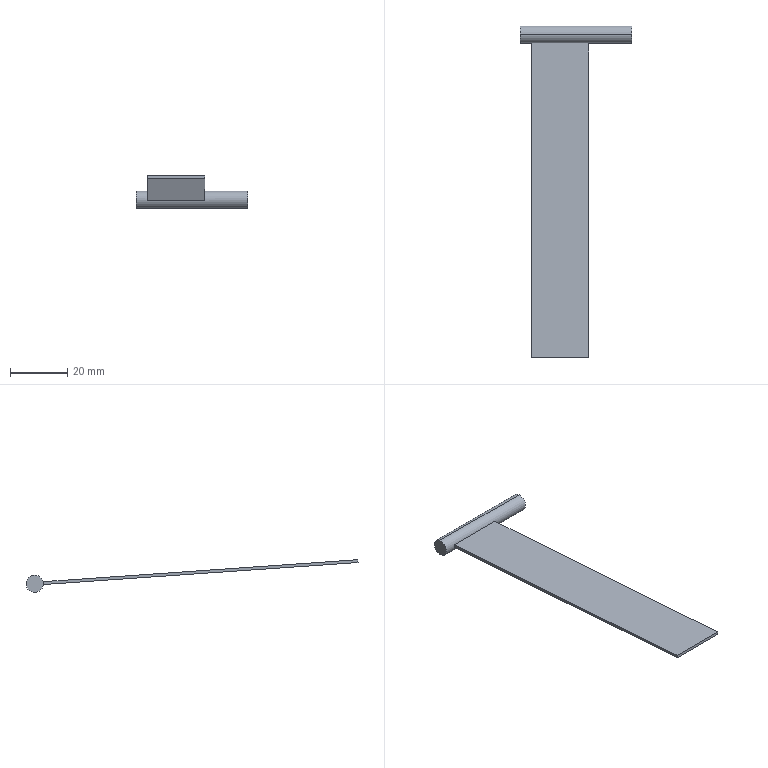Component | SolidWorks | OuterBagExpansionSheetMetalSidePlate-1 | 1 solid | 9 faces | box 39 x 115.72 x 11.36 mm | volume 3302 mm3 | plane 7 | cylinder 2 | commonest cylinder face diameters 6 x2
build123d program:
from build123d import *

# Parameters (mm, degrees)
SKETCH2_W                = 110
SKETCH2_H                = 20
BOSS_EXTRUDE1_DEPTH      = 1
BOSS_EXTRUDE2_DEPTH      = 4
BOSS_EXTRUDE2_DEPTH_BACK = 35
SKETCH3_R                = 3


with BuildPart() as part:
    # Sketch2 → Boss-Extrude1 (new body)
    with BuildSketch(Plane.XY):
        with Locations((-72.403, -7.81)):
            Rectangle(SKETCH2_W, SKETCH2_H)
    extrude(amount=BOSS_EXTRUDE1_DEPTH)

    # Sketch3 → Boss-Extrude2 (add, two sides: drawn at the far end of the back side and taken through both)
    with BuildSketch(Plane.XZ.offset(17.81).offset(-BOSS_EXTRUDE2_DEPTH_BACK)):
        with Locations(Location((-14.445, 0.5, 0), (0, 0, 270))):
            Circle(SKETCH3_R)
    extrude(amount=BOSS_EXTRUDE2_DEPTH + BOSS_EXTRUDE2_DEPTH_BACK)


solid = part.part

# Placed as in the assembly
solid = solid.moved(Location((-530.636, 26.871, 401.647), (176.009, 0, -90)))
STEP:
#1=COLOUR_RGB('',0.7922,0.8196,0.9333);
#2=FILL_AREA_STYLE_COLOUR('',#1);
#3=FILL_AREA_STYLE('',(#2));
#4=SURFACE_STYLE_FILL_AREA(#3);
#5=SURFACE_SIDE_STYLE('',(#4));
#6=SURFACE_STYLE_USAGE(.BOTH.,#5);
#7=PRESENTATION_STYLE_ASSIGNMENT((#6));
#8=CARTESIAN_POINT('',(-21.75,0.4975,15.951));
#9=VERTEX_POINT('',#8);
#10=CARTESIAN_POINT('',(-21.75,0.481,15.715));
#11=VERTEX_POINT('',#10);
#12=CARTESIAN_POINT('',(-21.75,0.4892,15.833));
#13=DIRECTION('',(-1.,0.,0.));
#14=DIRECTION('',(0.,0.0696,0.9976));
#15=AXIS2_PLACEMENT_3D('',#12,#13,#14);
#16=CIRCLE('',#15,0.1181);
#17=EDGE_CURVE('',#9,#11,#16,.T.);
#18=ORIENTED_EDGE('',*,*,#17,.F.);
#19=CARTESIAN_POINT('',(-20.214,0.4975,15.951));
#20=VERTEX_POINT('',#19);
#21=CARTESIAN_POINT('',(-21.75,0.4975,15.951));
#22=DIRECTION('',(1.,-0.,-0.));
#23=VECTOR('',#22,39.37);
#24=LINE('',#21,#23);
#25=EDGE_CURVE('',#9,#20,#24,.T.);
#26=ORIENTED_EDGE('',*,*,#25,.T.);
#27=CARTESIAN_POINT('',(-20.214,0.481,15.715));
#28=VERTEX_POINT('',#27);
#29=CARTESIAN_POINT('',(-20.214,0.4892,15.833));
#30=DIRECTION('',(-1.,0.,0.));
#31=DIRECTION('',(0.,0.0696,0.9976));
#32=AXIS2_PLACEMENT_3D('',#29,#30,#31);
#33=CIRCLE('',#32,0.1181);
#34=EDGE_CURVE('',#20,#28,#33,.T.);
#35=ORIENTED_EDGE('',*,*,#34,.T.);
#36=CARTESIAN_POINT('',(-21.75,0.481,15.715));
#37=DIRECTION('',(1.,-0.,-0.));
#38=VECTOR('',#37,39.37);
#39=LINE('',#36,#38);
#40=EDGE_CURVE('',#11,#28,#39,.T.);
#41=ORIENTED_EDGE('',*,*,#40,.F.);
#42=EDGE_LOOP('',(#18,#26,#35,#41));
#43=FACE_OUTER_BOUND('',#42,.T.);
#44=CARTESIAN_POINT('',(-21.75,0.4892,15.833));
#45=DIRECTION('',(1.,-0.,-0.));
#46=DIRECTION('',(0.,-0.0696,-0.9976));
#47=AXIS2_PLACEMENT_3D('',#44,#45,#46);
#48=CYLINDRICAL_SURFACE('',#47,0.1181);
#49=ADVANCED_FACE('',(#43),#48,.T.);
#50=CARTESIAN_POINT('',(-20.805,-3.946,16.162));
#51=VERTEX_POINT('',#50);
#52=CARTESIAN_POINT('',(-21.592,-3.946,16.162));
#53=VERTEX_POINT('',#52);
#54=CARTESIAN_POINT('',(-20.805,-3.946,16.162));
#55=DIRECTION('',(-1.,0.,0.));
#56=VECTOR('',#55,39.37);
#57=LINE('',#54,#56);
#58=EDGE_CURVE('',#51,#53,#57,.T.);
#59=ORIENTED_EDGE('',*,*,#58,.T.);
#60=CARTESIAN_POINT('',(-21.592,-3.949,16.123));
#61=VERTEX_POINT('',#60);
#62=CARTESIAN_POINT('',(-21.592,-3.949,16.123));
#63=DIRECTION('',(0.,0.0696,0.9976));
#64=VECTOR('',#63,39.37);
#65=LINE('',#62,#64);
#66=EDGE_CURVE('',#61,#53,#65,.T.);
#67=ORIENTED_EDGE('',*,*,#66,.F.);
#68=CARTESIAN_POINT('',(-20.805,-3.949,16.123));
#69=VERTEX_POINT('',#68);
#70=CARTESIAN_POINT('',(-20.805,-3.949,16.123));
#71=DIRECTION('',(-1.,0.,0.));
#72=VECTOR('',#71,39.37);
#73=LINE('',#70,#72);
#74=EDGE_CURVE('',#69,#61,#73,.T.);
#75=ORIENTED_EDGE('',*,*,#74,.F.);
#76=CARTESIAN_POINT('',(-20.805,-3.949,16.123));
#77=DIRECTION('',(0.,0.0696,0.9976));
#78=VECTOR('',#77,39.37);
#79=LINE('',#76,#78);
#80=EDGE_CURVE('',#69,#51,#79,.T.);
#81=ORIENTED_EDGE('',*,*,#80,.T.);
#82=EDGE_LOOP('',(#59,#67,#75,#81));
#83=FACE_OUTER_BOUND('',#82,.T.);
#84=CARTESIAN_POINT('',(-20.805,-3.949,16.123));
#85=DIRECTION('',(-0.,0.9976,-0.0696));
#86=DIRECTION('',(0.,0.0696,0.9976));
#87=AXIS2_PLACEMENT_3D('',#84,#85,#86);
#88=PLANE('',#87);
#89=ADVANCED_FACE('',(#83),#88,.F.);
#90=CARTESIAN_POINT('',(-21.592,0.3717,15.821));
#91=VERTEX_POINT('',#90);
#92=CARTESIAN_POINT('',(-21.592,0.3744,15.861));
#93=VERTEX_POINT('',#92);
#94=CARTESIAN_POINT('',(-21.592,0.4892,15.833));
#95=DIRECTION('',(-1.,0.,0.));
#96=DIRECTION('',(0.,-0.0696,-0.9976));
#97=AXIS2_PLACEMENT_3D('',#94,#95,#96);
#98=CIRCLE('',#97,0.1181);
#99=EDGE_CURVE('',#91,#93,#98,.T.);
#100=ORIENTED_EDGE('',*,*,#99,.F.);
#101=CARTESIAN_POINT('',(-21.592,-3.949,16.123));
#102=DIRECTION('',(-0.,0.9976,-0.0696));
#103=VECTOR('',#102,39.37);
#104=LINE('',#101,#103);
#105=EDGE_CURVE('',#61,#91,#104,.T.);
#106=ORIENTED_EDGE('',*,*,#105,.F.);
#107=ORIENTED_EDGE('',*,*,#66,.T.);
#108=CARTESIAN_POINT('',(-21.592,-3.946,16.162));
#109=DIRECTION('',(-0.,0.9976,-0.0696));
#110=VECTOR('',#109,39.37);
#111=LINE('',#108,#110);
#112=EDGE_CURVE('',#53,#93,#111,.T.);
#113=ORIENTED_EDGE('',*,*,#112,.T.);
#114=EDGE_LOOP('',(#100,#106,#107,#113));
#115=FACE_OUTER_BOUND('',#114,.T.);
#116=CARTESIAN_POINT('',(-21.592,-3.949,16.123));
#117=DIRECTION('',(1.,-0.,-0.));
#118=DIRECTION('',(-0.,-0.0696,-0.9976));
#119=AXIS2_PLACEMENT_3D('',#116,#117,#118);
#120=PLANE('',#119);
#121=ADVANCED_FACE('',(#115),#120,.F.);
#122=CARTESIAN_POINT('',(-20.805,0.3744,15.861));
#123=VERTEX_POINT('',#122);
#124=CARTESIAN_POINT('',(-20.805,0.3717,15.821));
#125=VERTEX_POINT('',#124);
#126=CARTESIAN_POINT('',(-20.805,0.4892,15.833));
#127=DIRECTION('',(1.,-0.,-0.));
#128=DIRECTION('',(0.,0.0696,0.9976));
#129=AXIS2_PLACEMENT_3D('',#126,#127,#128);
#130=CIRCLE('',#129,0.1181);
#131=EDGE_CURVE('',#123,#125,#130,.T.);
#132=ORIENTED_EDGE('',*,*,#131,.F.);
#133=CARTESIAN_POINT('',(-20.805,-3.946,16.162));
#134=DIRECTION('',(0.,-0.9976,0.0696));
#135=VECTOR('',#134,39.37);
#136=LINE('',#133,#135);
#137=EDGE_CURVE('',#123,#51,#136,.T.);
#138=ORIENTED_EDGE('',*,*,#137,.T.);
#139=ORIENTED_EDGE('',*,*,#80,.F.);
#140=CARTESIAN_POINT('',(-20.805,-3.949,16.123));
#141=DIRECTION('',(0.,-0.9976,0.0696));
#142=VECTOR('',#141,39.37);
#143=LINE('',#140,#142);
#144=EDGE_CURVE('',#125,#69,#143,.T.);
#145=ORIENTED_EDGE('',*,*,#144,.F.);
#146=EDGE_LOOP('',(#132,#138,#139,#145));
#147=FACE_OUTER_BOUND('',#146,.T.);
#148=CARTESIAN_POINT('',(-20.805,-3.949,16.123));
#149=DIRECTION('',(-1.,0.,0.));
#150=DIRECTION('',(0.,0.0696,0.9976));
#151=AXIS2_PLACEMENT_3D('',#148,#149,#150);
#152=PLANE('',#151);
#153=ADVANCED_FACE('',(#147),#152,.F.);
#154=ORIENTED_EDGE('',*,*,#74,.T.);
#155=ORIENTED_EDGE('',*,*,#105,.T.);
#156=CARTESIAN_POINT('',(-20.805,0.3717,15.821));
#157=DIRECTION('',(1.,0.,-0.));
#158=VECTOR('',#157,39.37);
#159=LINE('',#156,#158);
#160=EDGE_CURVE('',#91,#125,#159,.T.);
#161=ORIENTED_EDGE('',*,*,#160,.T.);
#162=ORIENTED_EDGE('',*,*,#144,.T.);
#163=EDGE_LOOP('',(#154,#155,#161,#162));
#164=FACE_OUTER_BOUND('',#163,.T.);
#165=CARTESIAN_POINT('',(-20.891,1.055,15.774));
#166=DIRECTION('',(-0.,-0.0696,-0.9976));
#167=DIRECTION('',(-0.,0.9976,-0.0696));
#168=AXIS2_PLACEMENT_3D('',#165,#166,#167);
#169=PLANE('',#168);
#170=ADVANCED_FACE('',(#164),#169,.T.);
#171=ORIENTED_EDGE('',*,*,#58,.F.);
#172=ORIENTED_EDGE('',*,*,#137,.F.);
#173=CARTESIAN_POINT('',(-20.805,0.3744,15.861));
#174=DIRECTION('',(1.,0.,-0.));
#175=VECTOR('',#174,39.37);
#176=LINE('',#173,#175);
#177=EDGE_CURVE('',#93,#123,#176,.T.);
#178=ORIENTED_EDGE('',*,*,#177,.F.);
#179=ORIENTED_EDGE('',*,*,#112,.F.);
#180=EDGE_LOOP('',(#171,#172,#178,#179));
#181=FACE_OUTER_BOUND('',#180,.T.);
#182=CARTESIAN_POINT('',(-20.891,1.058,15.813));
#183=DIRECTION('',(-0.,-0.0696,-0.9976));
#184=DIRECTION('',(-0.,0.9976,-0.0696));
#185=AXIS2_PLACEMENT_3D('',#182,#183,#184);
#186=PLANE('',#185);
#187=ADVANCED_FACE('',(#181),#186,.F.);
#188=ORIENTED_EDGE('',*,*,#25,.F.);
#189=CARTESIAN_POINT('',(-21.75,0.4892,15.833));
#190=DIRECTION('',(-1.,0.,0.));
#191=DIRECTION('',(0.,0.0696,0.9976));
#192=AXIS2_PLACEMENT_3D('',#189,#190,#191);
#193=CIRCLE('',#192,0.1181);
#194=EDGE_CURVE('',#11,#9,#193,.T.);
#195=ORIENTED_EDGE('',*,*,#194,.F.);
#196=ORIENTED_EDGE('',*,*,#40,.T.);
#197=CARTESIAN_POINT('',(-20.214,0.4892,15.833));
#198=DIRECTION('',(-1.,0.,0.));
#199=DIRECTION('',(0.,0.0696,0.9976));
#200=AXIS2_PLACEMENT_3D('',#197,#198,#199);
#201=CIRCLE('',#200,0.1181);
#202=EDGE_CURVE('',#28,#20,#201,.T.);
#203=ORIENTED_EDGE('',*,*,#202,.T.);
#204=EDGE_LOOP('',(#188,#195,#196,#203));
#205=FACE_OUTER_BOUND('',#204,.T.);
#206=ORIENTED_EDGE('',*,*,#160,.F.);
#207=ORIENTED_EDGE('',*,*,#99,.T.);
#208=ORIENTED_EDGE('',*,*,#177,.T.);
#209=ORIENTED_EDGE('',*,*,#131,.T.);
#210=EDGE_LOOP('',(#206,#207,#208,#209));
#211=FACE_BOUND('',#210,.T.);
#212=CARTESIAN_POINT('',(-21.75,0.4892,15.833));
#213=DIRECTION('',(1.,-0.,-0.));
#214=DIRECTION('',(0.,-0.0696,-0.9976));
#215=AXIS2_PLACEMENT_3D('',#212,#213,#214);
#216=CYLINDRICAL_SURFACE('',#215,0.1181);
#217=ADVANCED_FACE('',(#205,#211),#216,.T.);
#218=ORIENTED_EDGE('',*,*,#194,.T.);
#219=ORIENTED_EDGE('',*,*,#17,.T.);
#220=EDGE_LOOP('',(#218,#219));
#221=FACE_OUTER_BOUND('',#220,.T.);
#222=CARTESIAN_POINT('',(-21.75,0.4892,15.833));
#223=DIRECTION('',(-1.,0.,0.));
#224=DIRECTION('',(0.,0.0696,0.9976));
#225=AXIS2_PLACEMENT_3D('',#222,#223,#224);
#226=PLANE('',#225);
#227=ADVANCED_FACE('',(#221),#226,.T.);
#228=ORIENTED_EDGE('',*,*,#202,.F.);
#229=ORIENTED_EDGE('',*,*,#34,.F.);
#230=EDGE_LOOP('',(#228,#229));
#231=FACE_OUTER_BOUND('',#230,.T.);
#232=CARTESIAN_POINT('',(-20.214,0.4892,15.833));
#233=DIRECTION('',(-1.,0.,0.));
#234=DIRECTION('',(0.,0.0696,0.9976));
#235=AXIS2_PLACEMENT_3D('',#232,#233,#234);
#236=PLANE('',#235);
#237=ADVANCED_FACE('',(#231),#236,.F.);
#238=CLOSED_SHELL('',(#49,#89,#121,#153,#170,#187,#217,#227,#237));
#239=MANIFOLD_SOLID_BREP('',#238);
#240=STYLED_ITEM('',(#7),#239);
#241=PRESENTATION_LAYER_ASSIGNMENT('','',(#240));
#242=(LENGTH_UNIT()NAMED_UNIT(*)SI_UNIT($,.METRE.));
#243=LENGTH_MEASURE_WITH_UNIT(LENGTH_MEASURE(0.0254),#242);
#244=DIMENSIONAL_EXPONENTS(1.,0.,0.,0.,0.,0.,0.);
#245=(CONVERSION_BASED_UNIT('',#243)LENGTH_UNIT()NAMED_UNIT(#244));
#246=UNCERTAINTY_MEASURE_WITH_UNIT(LENGTH_MEASURE(0.00001),#245,'','');
#247=(NAMED_UNIT(*)PLANE_ANGLE_UNIT()SI_UNIT($,.RADIAN.));
#248=(NAMED_UNIT(*)SI_UNIT($,.STERADIAN.)SOLID_ANGLE_UNIT());
#249=(GEOMETRIC_REPRESENTATION_CONTEXT(3)GLOBAL_UNCERTAINTY_ASSIGNED_CONTEXT((#246))GLOBAL_UNIT_ASSIGNED_CONTEXT((#245,#247,#248))REPRESENTATION_CONTEXT('',''));
#250=MECHANICAL_DESIGN_GEOMETRIC_PRESENTATION_REPRESENTATION('',(#240),#249);
#251=CARTESIAN_POINT('',(0.,0.,0.));
#252=DIRECTION('',(0.,0.,1.));
#253=DIRECTION('',(1.,0.,0.));
#254=AXIS2_PLACEMENT_3D('',#251,#252,#253);
#255=(LENGTH_UNIT()NAMED_UNIT(*)SI_UNIT($,.METRE.));
#256=LENGTH_MEASURE_WITH_UNIT(LENGTH_MEASURE(0.0254),#255);
#257=DIMENSIONAL_EXPONENTS(1.,0.,0.,0.,0.,0.,0.);
#258=(CONVERSION_BASED_UNIT('',#256)LENGTH_UNIT()NAMED_UNIT(#257));
#259=UNCERTAINTY_MEASURE_WITH_UNIT(LENGTH_MEASURE(0.00001),#258,'','');
#260=(NAMED_UNIT(*)PLANE_ANGLE_UNIT()SI_UNIT($,.RADIAN.));
#261=(NAMED_UNIT(*)SI_UNIT($,.STERADIAN.)SOLID_ANGLE_UNIT());
#262=(GEOMETRIC_REPRESENTATION_CONTEXT(3)GLOBAL_UNCERTAINTY_ASSIGNED_CONTEXT((#259))GLOBAL_UNIT_ASSIGNED_CONTEXT((#258,#260,#261))REPRESENTATION_CONTEXT('',''));
#263=ADVANCED_BREP_SHAPE_REPRESENTATION('',(#239,#254),#262);